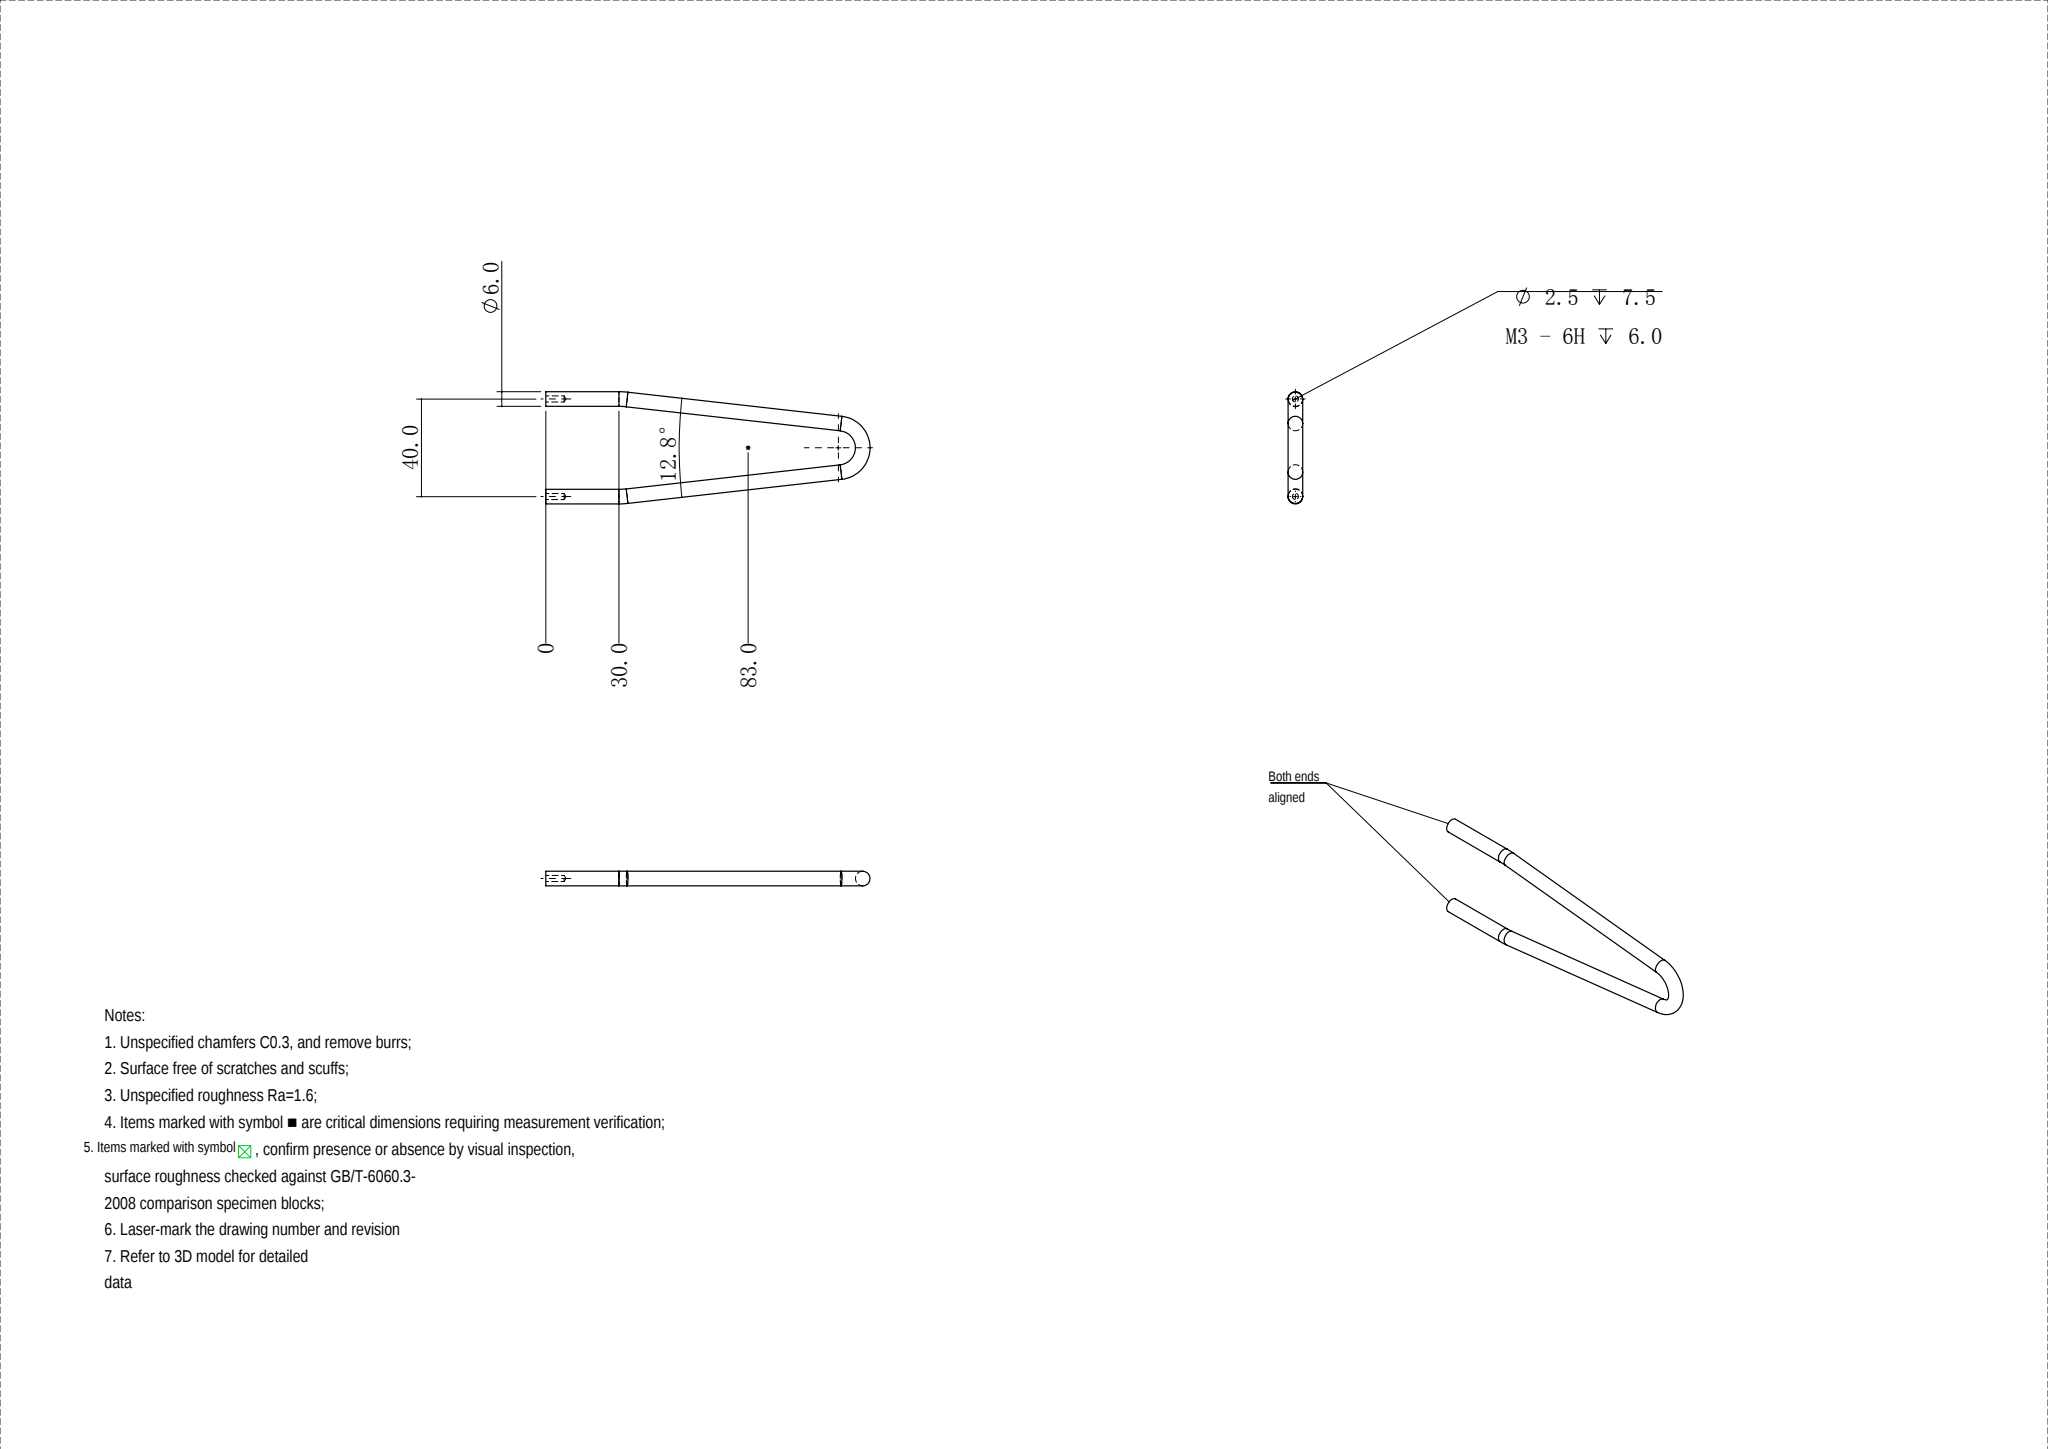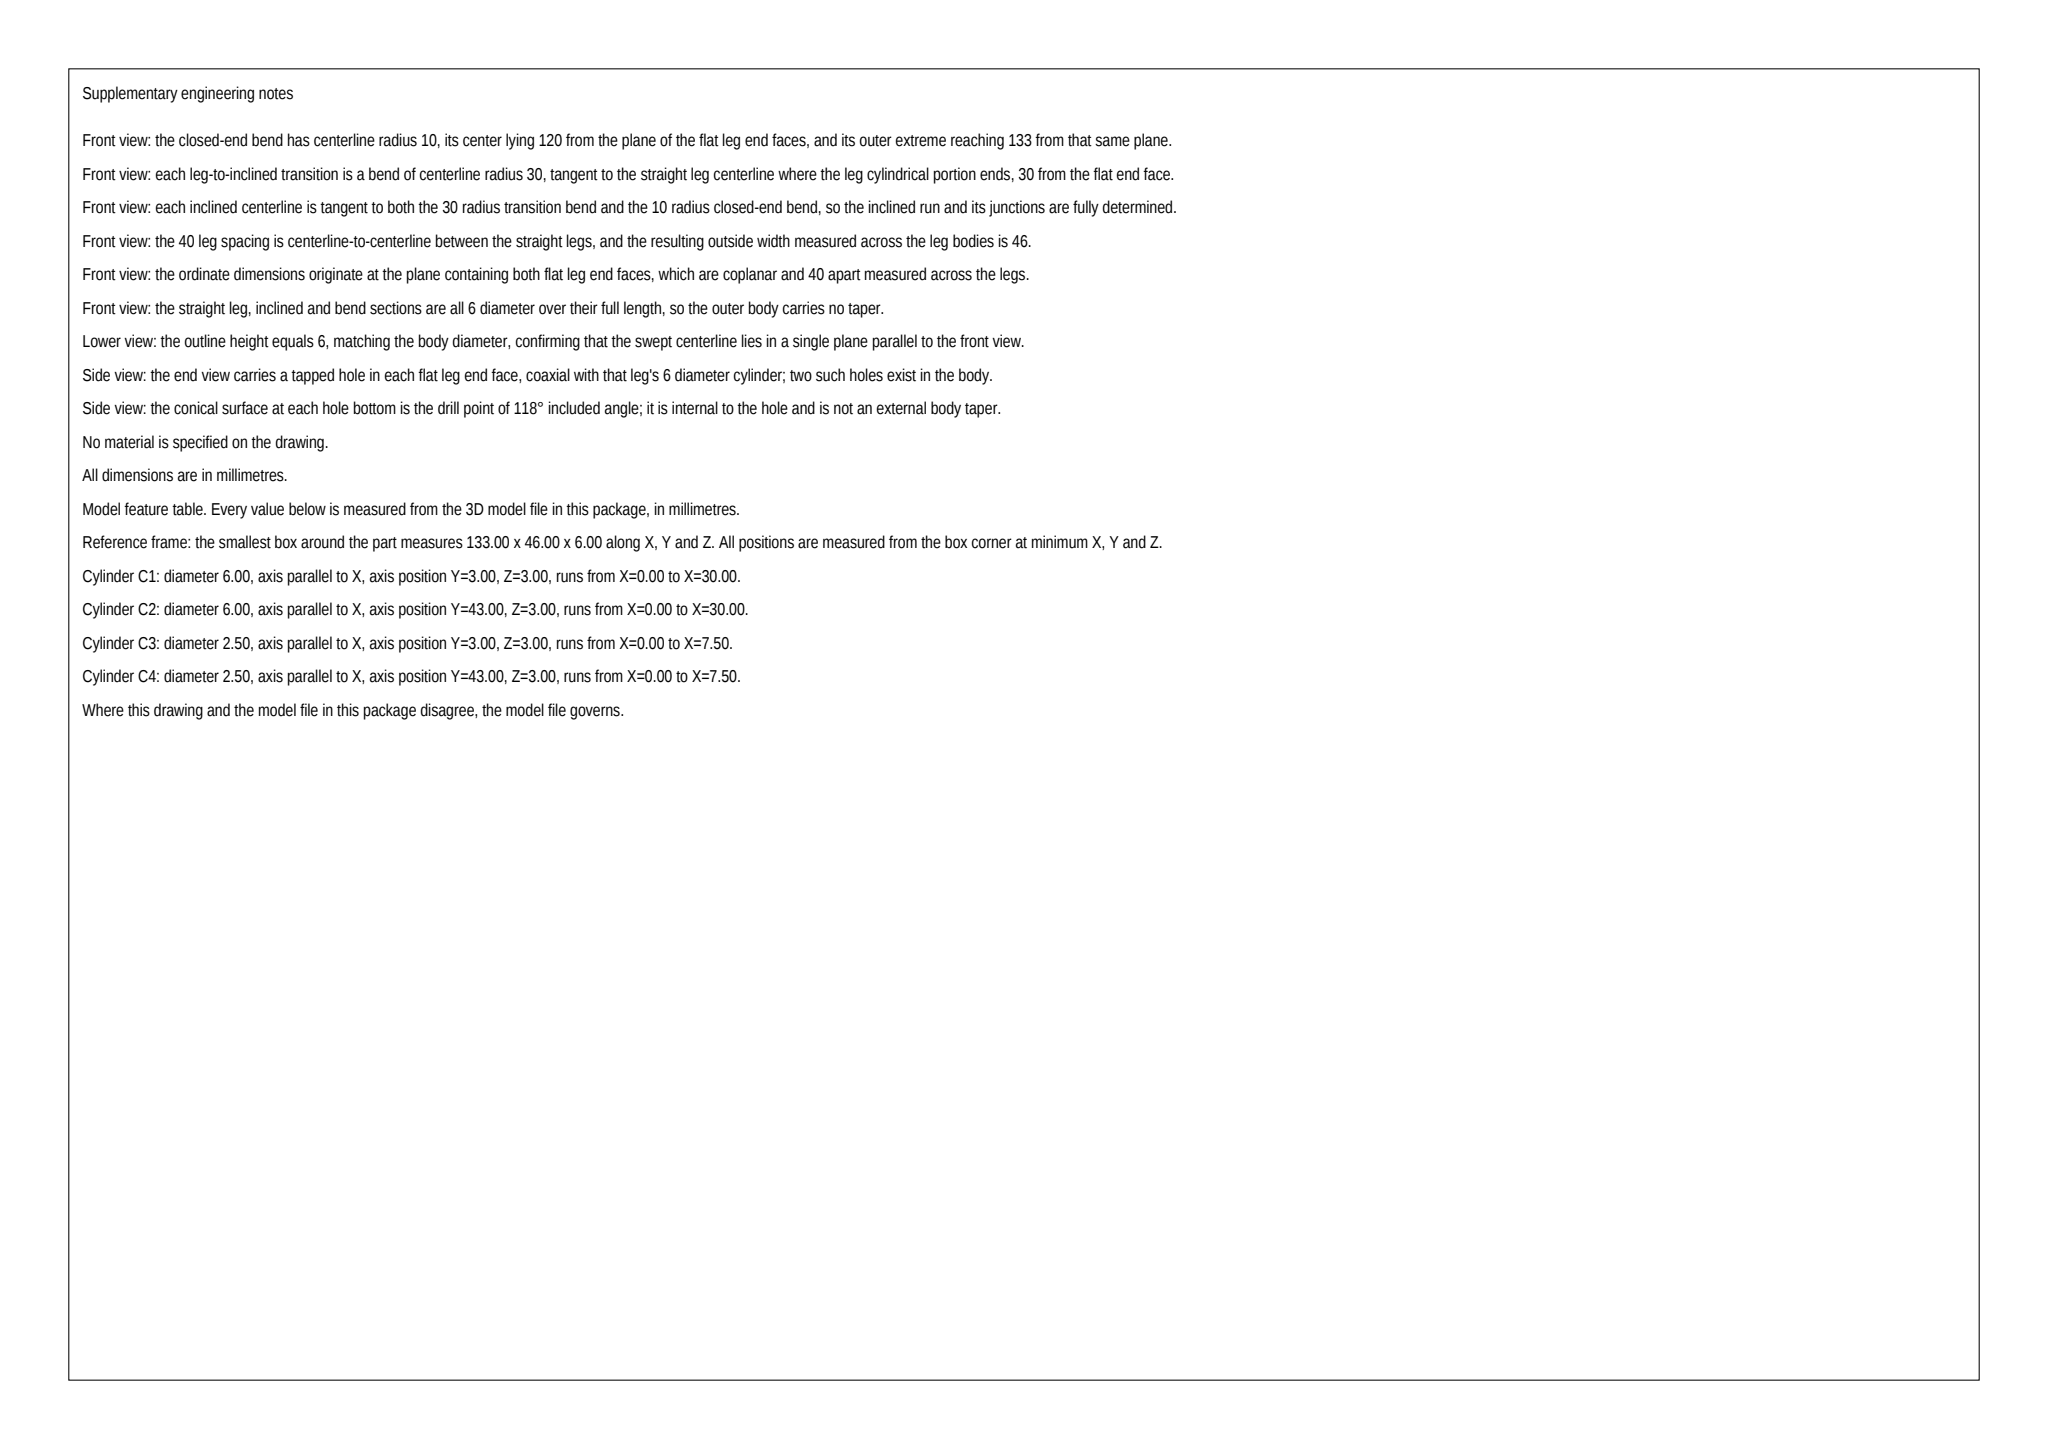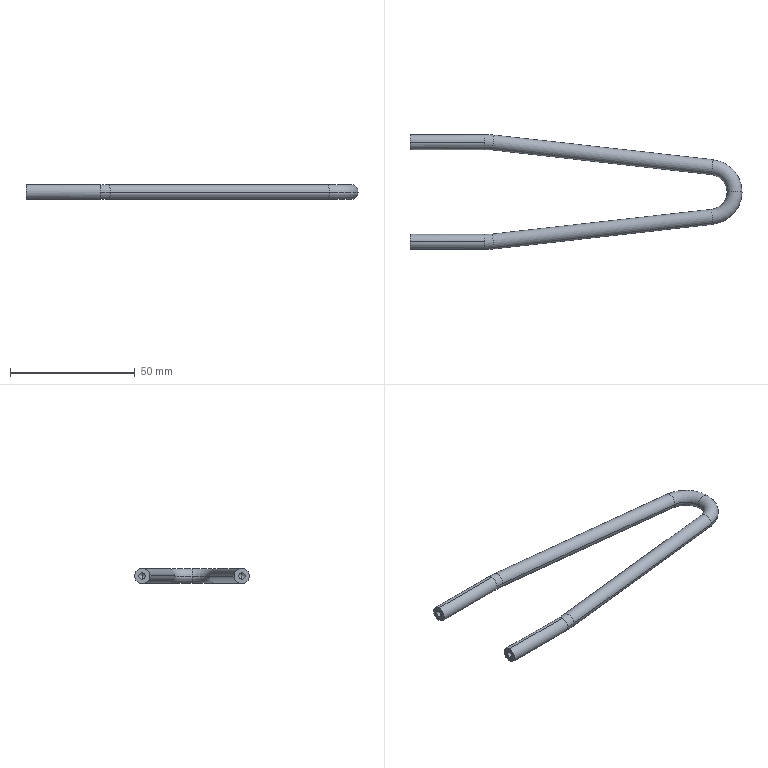Part | SolidWorks | mm | 1 solid | 26 faces | box 133 x 46 x 6 mm | volume 7630 mm3 | cylinder 12 | torus 8 | cone 4 | plane 2 | commonest cylinder face diameters 6 x8 2.5 x4
Drawing notes:
2X Ø2.5 DP 7.5, M3 - 6H DP 6.0 | from the solid: cylinders dia 2.5 axis x at y=3.05 and y=43.05, len 7.5, count 2 each (one per leg end)
Ø2.5/M3 HOLES COAX W/ Ø6.0 LEGS, IN END FACES AT STA 0 | from the solid: Ø2.5 holes share y=3.05/43.05, z=3.0 with Ø6.0 leg cylinders; axis plane x=0.0 end faces
40.0 IS CL-TO-CL OF Ø6.0 LEGS | from the solid: Ø6.0 leg axes at y=3.05 and y=43.05 -> 40.0 between centerlines
2X R30 TAN AT STA 30.0; 88.43 STRAIGHT TO R10 TANGENT | from the solid: Ø6.0 straight legs len 30.0 from x=0; angled Ø6.0 cylinders len 88.43 (y=3.24, y=32.99)
build123d program:
from build123d import *

# Parameters (mm, degrees)
SWEEP1_PROFILE_R      = 3
M3_TAPPED_HOLE1_D     = 2.5
M3_TAPPED_HOLE1_DEPTH = 7.5
M3_TAPPED_HOLE1_TIP   = 0.7511


with BuildPart() as part:
    # Sweep1: sweep along a curve in space
    with BuildLine() as sweep1_path:
        Line((0, 0, 0), (30, 0, 0))
        ThreePointArc((30, 0, 0), (31.68, -0.04706, 0), (33.354, -0.1881, 0))
        Line((33.354, -0.1881, 0), (121.118, -10.063, 0))
        ThreePointArc((121.118, -10.063, 0), (130, -20, 0), (121.118, -29.937, 0))
        Line((33.354, -39.812, 0), (121.118, -29.937, 0))
        ThreePointArc((30, -40, 0), (31.68, -39.953, 0), (33.354, -39.812, 0))
        Line((0, -40, 0), (30, -40, 0))
    # Sweep1 profile (on start of the path) → Sweep1 (sweep)
    with BuildSketch(Plane(origin=(0, 0, 0), x_dir=(0, 0, 1), z_dir=(1, 0, 0))):
        Circle(SWEEP1_PROFILE_R)
    sweep(path=sweep1_path.line)

    # M3 Tapped Hole1
    with Locations(Plane.ZY):
        with Locations((0, 0), (0, -40)):
            Hole(M3_TAPPED_HOLE1_D / 2, depth=M3_TAPPED_HOLE1_DEPTH)
            with Locations((0, 0, -(M3_TAPPED_HOLE1_DEPTH + M3_TAPPED_HOLE1_TIP / 2))):  # 118° drill point
                Cone(0, M3_TAPPED_HOLE1_D / 2, M3_TAPPED_HOLE1_TIP, mode=Mode.SUBTRACT)


solid = part.part
STEP:
#1=CARTESIAN_POINT('',(33.019,-3.169,0.));
#2=VERTEX_POINT('',#1);
#3=CARTESIAN_POINT('',(33.69,2.793,0.));
#4=VERTEX_POINT('',#3);
#5=CARTESIAN_POINT('',(33.354,-0.1881,0.));
#6=DIRECTION('',(-0.9937,0.1118,0.));
#7=DIRECTION('',(0.,0.,-1.));
#8=AXIS2_PLACEMENT_3D('',#5,#6,#7);
#9=CIRCLE('',#8,3.);
#10=EDGE_CURVE('',#2,#4,#9,.T.);
#11=ORIENTED_EDGE('',*,*,#10,.T.);
#12=CARTESIAN_POINT('',(30.,3.,0.));
#13=VERTEX_POINT('',#12);
#14=CARTESIAN_POINT('',(30.,-30.,0.));
#15=DIRECTION('',(0.,-0.,1.));
#16=DIRECTION('',(0.,-1.,-0.));
#17=AXIS2_PLACEMENT_3D('',#14,#15,#16);
#18=CIRCLE('',#17,33.);
#19=EDGE_CURVE('',#4,#13,#18,.T.);
#20=ORIENTED_EDGE('',*,*,#19,.T.);
#21=CARTESIAN_POINT('',(30.,0.,3.));
#22=VERTEX_POINT('',#21);
#23=CARTESIAN_POINT('',(30.,0.,0.));
#24=DIRECTION('',(-1.,-0.,0.));
#25=DIRECTION('',(0.,0.,-1.));
#26=AXIS2_PLACEMENT_3D('',#23,#24,#25);
#27=CIRCLE('',#26,3.);
#28=EDGE_CURVE('',#22,#13,#27,.T.);
#29=ORIENTED_EDGE('',*,*,#28,.F.);
#30=CARTESIAN_POINT('',(30.,-3.,0.));
#31=VERTEX_POINT('',#30);
#32=CARTESIAN_POINT('',(30.,0.,0.));
#33=DIRECTION('',(-1.,-0.,0.));
#34=DIRECTION('',(0.,0.,-1.));
#35=AXIS2_PLACEMENT_3D('',#32,#33,#34);
#36=CIRCLE('',#35,3.);
#37=EDGE_CURVE('',#31,#22,#36,.T.);
#38=ORIENTED_EDGE('',*,*,#37,.F.);
#39=CARTESIAN_POINT('',(30.,-30.,0.));
#40=DIRECTION('',(0.,-0.,1.));
#41=DIRECTION('',(0.,-1.,-0.));
#42=AXIS2_PLACEMENT_3D('',#39,#40,#41);
#43=CIRCLE('',#42,27.);
#44=EDGE_CURVE('',#2,#31,#43,.T.);
#45=ORIENTED_EDGE('',*,*,#44,.F.);
#46=EDGE_LOOP('',(#11,#20,#29,#38,#45));
#47=FACE_OUTER_BOUND('',#46,.T.);
#48=CARTESIAN_POINT('',(30.,-30.,0.));
#49=DIRECTION('',(0.,-0.,1.));
#50=DIRECTION('',(0.,-1.,-0.));
#51=AXIS2_PLACEMENT_3D('',#48,#49,#50);
#52=TOROIDAL_SURFACE('',#51,30.,3.);
#53=ADVANCED_FACE('',(#47),#52,.T.);
#54=CARTESIAN_POINT('',(133.,-20.,0.));
#55=VERTEX_POINT('',#54);
#56=CARTESIAN_POINT('',(127.,-20.,-0.));
#57=VERTEX_POINT('',#56);
#58=CARTESIAN_POINT('',(130.,-20.,0.));
#59=DIRECTION('',(0.,-1.,0.));
#60=DIRECTION('',(0.,0.,-1.));
#61=AXIS2_PLACEMENT_3D('',#58,#59,#60);
#62=CIRCLE('',#61,3.);
#63=EDGE_CURVE('',#55,#57,#62,.T.);
#64=ORIENTED_EDGE('',*,*,#63,.F.);
#65=CARTESIAN_POINT('',(121.454,-7.082,0.));
#66=VERTEX_POINT('',#65);
#67=CARTESIAN_POINT('',(120.,-20.,0.));
#68=DIRECTION('',(0.,0.,1.));
#69=DIRECTION('',(1.,0.,0.));
#70=AXIS2_PLACEMENT_3D('',#67,#68,#69);
#71=CIRCLE('',#70,13.);
#72=EDGE_CURVE('',#55,#66,#71,.T.);
#73=ORIENTED_EDGE('',*,*,#72,.T.);
#74=CARTESIAN_POINT('',(120.783,-13.044,0.));
#75=VERTEX_POINT('',#74);
#76=CARTESIAN_POINT('',(121.118,-10.063,0.));
#77=DIRECTION('',(-0.9937,0.1118,0.));
#78=DIRECTION('',(0.,0.,-1.));
#79=AXIS2_PLACEMENT_3D('',#76,#77,#78);
#80=CIRCLE('',#79,3.);
#81=EDGE_CURVE('',#75,#66,#80,.T.);
#82=ORIENTED_EDGE('',*,*,#81,.F.);
#83=CARTESIAN_POINT('',(120.,-20.,-0.));
#84=DIRECTION('',(0.,0.,1.));
#85=DIRECTION('',(1.,0.,0.));
#86=AXIS2_PLACEMENT_3D('',#83,#84,#85);
#87=CIRCLE('',#86,7.);
#88=EDGE_CURVE('',#57,#75,#87,.T.);
#89=ORIENTED_EDGE('',*,*,#88,.F.);
#90=EDGE_LOOP('',(#64,#73,#82,#89));
#91=FACE_OUTER_BOUND('',#90,.T.);
#92=CARTESIAN_POINT('',(120.,-20.,0.));
#93=DIRECTION('',(0.,0.,1.));
#94=DIRECTION('',(1.,0.,0.));
#95=AXIS2_PLACEMENT_3D('',#92,#93,#94);
#96=TOROIDAL_SURFACE('',#95,10.,3.);
#97=ADVANCED_FACE('',(#91),#96,.T.);
#98=CARTESIAN_POINT('',(30.,-40.,3.));
#99=VERTEX_POINT('',#98);
#100=CARTESIAN_POINT('',(30.,-43.,0.));
#101=VERTEX_POINT('',#100);
#102=CARTESIAN_POINT('',(30.,-40.,-0.));
#103=DIRECTION('',(1.,0.,-0.));
#104=DIRECTION('',(-0.,0.,-1.));
#105=AXIS2_PLACEMENT_3D('',#102,#103,#104);
#106=CIRCLE('',#105,3.);
#107=EDGE_CURVE('',#99,#101,#106,.T.);
#108=ORIENTED_EDGE('',*,*,#107,.T.);
#109=CARTESIAN_POINT('',(33.69,-42.793,0.));
#110=VERTEX_POINT('',#109);
#111=CARTESIAN_POINT('',(30.,-10.,0.));
#112=DIRECTION('',(0.,-0.,1.));
#113=DIRECTION('',(1.,0.,-0.));
#114=AXIS2_PLACEMENT_3D('',#111,#112,#113);
#115=CIRCLE('',#114,33.);
#116=EDGE_CURVE('',#101,#110,#115,.T.);
#117=ORIENTED_EDGE('',*,*,#116,.T.);
#118=CARTESIAN_POINT('',(33.019,-36.831,0.));
#119=VERTEX_POINT('',#118);
#120=CARTESIAN_POINT('',(33.354,-39.812,0.));
#121=DIRECTION('',(0.9937,0.1118,-0.));
#122=DIRECTION('',(0.,0.,-1.));
#123=AXIS2_PLACEMENT_3D('',#120,#121,#122);
#124=CIRCLE('',#123,3.);
#125=EDGE_CURVE('',#119,#110,#124,.T.);
#126=ORIENTED_EDGE('',*,*,#125,.F.);
#127=CARTESIAN_POINT('',(30.,-37.,0.));
#128=VERTEX_POINT('',#127);
#129=CARTESIAN_POINT('',(30.,-10.,0.));
#130=DIRECTION('',(0.,-0.,1.));
#131=DIRECTION('',(1.,0.,-0.));
#132=AXIS2_PLACEMENT_3D('',#129,#130,#131);
#133=CIRCLE('',#132,27.);
#134=EDGE_CURVE('',#128,#119,#133,.T.);
#135=ORIENTED_EDGE('',*,*,#134,.F.);
#136=CARTESIAN_POINT('',(30.,-40.,-0.));
#137=DIRECTION('',(1.,0.,-0.));
#138=DIRECTION('',(-0.,0.,-1.));
#139=AXIS2_PLACEMENT_3D('',#136,#137,#138);
#140=CIRCLE('',#139,3.);
#141=EDGE_CURVE('',#128,#99,#140,.T.);
#142=ORIENTED_EDGE('',*,*,#141,.T.);
#143=EDGE_LOOP('',(#108,#117,#126,#135,#142));
#144=FACE_OUTER_BOUND('',#143,.T.);
#145=CARTESIAN_POINT('',(30.,-10.,0.));
#146=DIRECTION('',(0.,-0.,1.));
#147=DIRECTION('',(1.,0.,-0.));
#148=AXIS2_PLACEMENT_3D('',#145,#146,#147);
#149=TOROIDAL_SURFACE('',#148,30.,3.);
#150=ADVANCED_FACE('',(#144),#149,.T.);
#151=CARTESIAN_POINT('',(120.783,-26.956,0.));
#152=VERTEX_POINT('',#151);
#153=CARTESIAN_POINT('',(121.454,-32.918,0.));
#154=VERTEX_POINT('',#153);
#155=CARTESIAN_POINT('',(121.118,-29.937,0.));
#156=DIRECTION('',(0.9937,0.1118,0.));
#157=DIRECTION('',(0.,0.,-1.));
#158=AXIS2_PLACEMENT_3D('',#155,#156,#157);
#159=CIRCLE('',#158,3.);
#160=EDGE_CURVE('',#152,#154,#159,.T.);
#161=ORIENTED_EDGE('',*,*,#160,.T.);
#162=CARTESIAN_POINT('',(120.,-20.,0.));
#163=DIRECTION('',(0.,0.,1.));
#164=DIRECTION('',(1.,0.,0.));
#165=AXIS2_PLACEMENT_3D('',#162,#163,#164);
#166=CIRCLE('',#165,13.);
#167=EDGE_CURVE('',#154,#55,#166,.T.);
#168=ORIENTED_EDGE('',*,*,#167,.T.);
#169=ORIENTED_EDGE('',*,*,#63,.T.);
#170=CARTESIAN_POINT('',(120.,-20.,-0.));
#171=DIRECTION('',(0.,0.,1.));
#172=DIRECTION('',(1.,0.,0.));
#173=AXIS2_PLACEMENT_3D('',#170,#171,#172);
#174=CIRCLE('',#173,7.);
#175=EDGE_CURVE('',#152,#57,#174,.T.);
#176=ORIENTED_EDGE('',*,*,#175,.F.);
#177=EDGE_LOOP('',(#161,#168,#169,#176));
#178=FACE_OUTER_BOUND('',#177,.T.);
#179=CARTESIAN_POINT('',(120.,-20.,0.));
#180=DIRECTION('',(0.,0.,1.));
#181=DIRECTION('',(1.,0.,0.));
#182=AXIS2_PLACEMENT_3D('',#179,#180,#181);
#183=TOROIDAL_SURFACE('',#182,10.,3.);
#184=ADVANCED_FACE('',(#178),#183,.T.);
#185=CARTESIAN_POINT('',(7.5,0.,-1.25));
#186=VERTEX_POINT('',#185);
#187=CARTESIAN_POINT('',(7.5,0.,1.25));
#188=VERTEX_POINT('',#187);
#189=CARTESIAN_POINT('',(7.5,0.,0.));
#190=DIRECTION('',(-1.,0.,0.));
#191=DIRECTION('',(0.,0.,1.));
#192=AXIS2_PLACEMENT_3D('',#189,#190,#191);
#193=CIRCLE('',#192,1.25);
#194=EDGE_CURVE('',#186,#188,#193,.T.);
#195=ORIENTED_EDGE('',*,*,#194,.F.);
#196=CARTESIAN_POINT('',(-0.,0.,-1.25));
#197=VERTEX_POINT('',#196);
#198=CARTESIAN_POINT('',(0.,0.,-1.25));
#199=DIRECTION('',(-1.,0.,0.));
#200=VECTOR('',#199,1000.);
#201=LINE('',#198,#200);
#202=EDGE_CURVE('',#186,#197,#201,.T.);
#203=ORIENTED_EDGE('',*,*,#202,.T.);
#204=CARTESIAN_POINT('',(-0.,0.,1.25));
#205=VERTEX_POINT('',#204);
#206=CARTESIAN_POINT('',(-0.,0.,0.));
#207=DIRECTION('',(-1.,0.,0.));
#208=DIRECTION('',(0.,0.,1.));
#209=AXIS2_PLACEMENT_3D('',#206,#207,#208);
#210=CIRCLE('',#209,1.25);
#211=EDGE_CURVE('',#197,#205,#210,.T.);
#212=ORIENTED_EDGE('',*,*,#211,.T.);
#213=CARTESIAN_POINT('',(0.,0.,1.25));
#214=DIRECTION('',(-1.,0.,0.));
#215=VECTOR('',#214,1000.);
#216=LINE('',#213,#215);
#217=EDGE_CURVE('',#188,#205,#216,.T.);
#218=ORIENTED_EDGE('',*,*,#217,.F.);
#219=EDGE_LOOP('',(#195,#203,#212,#218));
#220=FACE_OUTER_BOUND('',#219,.T.);
#221=CARTESIAN_POINT('',(0.,0.,0.));
#222=DIRECTION('',(-1.,0.,0.));
#223=DIRECTION('',(0.,0.,1.));
#224=AXIS2_PLACEMENT_3D('',#221,#222,#223);
#225=CYLINDRICAL_SURFACE('',#224,1.25);
#226=ADVANCED_FACE('',(#220),#225,.F.);
#227=CARTESIAN_POINT('',(8.251,-0.,0.));
#228=VERTEX_POINT('',#227);
#229=CARTESIAN_POINT('',(7.5,0.,1.25));
#230=DIRECTION('',(-0.515,0.,0.8572));
#231=VECTOR('',#230,1000.);
#232=LINE('',#229,#231);
#233=EDGE_CURVE('',#228,#188,#232,.T.);
#234=ORIENTED_EDGE('',*,*,#233,.F.);
#235=CARTESIAN_POINT('',(7.5,0.,-1.25));
#236=DIRECTION('',(-0.515,0.,-0.8572));
#237=VECTOR('',#236,1000.);
#238=LINE('',#235,#237);
#239=EDGE_CURVE('',#228,#186,#238,.T.);
#240=ORIENTED_EDGE('',*,*,#239,.T.);
#241=ORIENTED_EDGE('',*,*,#194,.T.);
#242=EDGE_LOOP('',(#234,#240,#241));
#243=FACE_OUTER_BOUND('',#242,.T.);
#244=CARTESIAN_POINT('',(7.5,0.,0.));
#245=DIRECTION('',(-1.,0.,0.));
#246=DIRECTION('',(0.,0.,1.));
#247=AXIS2_PLACEMENT_3D('',#244,#245,#246);
#248=CONICAL_SURFACE('',#247,1.25,1.03);
#249=ADVANCED_FACE('',(#243),#248,.F.);
#250=CARTESIAN_POINT('',(7.5,-40.,-1.25));
#251=VERTEX_POINT('',#250);
#252=CARTESIAN_POINT('',(7.5,-40.,1.25));
#253=VERTEX_POINT('',#252);
#254=CARTESIAN_POINT('',(7.5,-40.,-0.));
#255=DIRECTION('',(-1.,0.,0.));
#256=DIRECTION('',(0.,0.,1.));
#257=AXIS2_PLACEMENT_3D('',#254,#255,#256);
#258=CIRCLE('',#257,1.25);
#259=EDGE_CURVE('',#251,#253,#258,.T.);
#260=ORIENTED_EDGE('',*,*,#259,.F.);
#261=CARTESIAN_POINT('',(-0.,-40.,-1.25));
#262=VERTEX_POINT('',#261);
#263=CARTESIAN_POINT('',(0.,-40.,-1.25));
#264=DIRECTION('',(-1.,0.,0.));
#265=VECTOR('',#264,1000.);
#266=LINE('',#263,#265);
#267=EDGE_CURVE('',#251,#262,#266,.T.);
#268=ORIENTED_EDGE('',*,*,#267,.T.);
#269=CARTESIAN_POINT('',(-0.,-40.,1.25));
#270=VERTEX_POINT('',#269);
#271=CARTESIAN_POINT('',(-0.,-40.,-0.));
#272=DIRECTION('',(-1.,0.,0.));
#273=DIRECTION('',(0.,0.,1.));
#274=AXIS2_PLACEMENT_3D('',#271,#272,#273);
#275=CIRCLE('',#274,1.25);
#276=EDGE_CURVE('',#262,#270,#275,.T.);
#277=ORIENTED_EDGE('',*,*,#276,.T.);
#278=CARTESIAN_POINT('',(0.,-40.,1.25));
#279=DIRECTION('',(-1.,0.,0.));
#280=VECTOR('',#279,1000.);
#281=LINE('',#278,#280);
#282=EDGE_CURVE('',#253,#270,#281,.T.);
#283=ORIENTED_EDGE('',*,*,#282,.F.);
#284=EDGE_LOOP('',(#260,#268,#277,#283));
#285=FACE_OUTER_BOUND('',#284,.T.);
#286=CARTESIAN_POINT('',(0.,-40.,-0.));
#287=DIRECTION('',(-1.,0.,0.));
#288=DIRECTION('',(0.,0.,1.));
#289=AXIS2_PLACEMENT_3D('',#286,#287,#288);
#290=CYLINDRICAL_SURFACE('',#289,1.25);
#291=ADVANCED_FACE('',(#285),#290,.F.);
#292=CARTESIAN_POINT('',(8.251,-40.,-0.));
#293=VERTEX_POINT('',#292);
#294=CARTESIAN_POINT('',(7.5,-40.,1.25));
#295=DIRECTION('',(-0.515,0.,0.8572));
#296=VECTOR('',#295,1000.);
#297=LINE('',#294,#296);
#298=EDGE_CURVE('',#293,#253,#297,.T.);
#299=ORIENTED_EDGE('',*,*,#298,.F.);
#300=CARTESIAN_POINT('',(7.5,-40.,-1.25));
#301=DIRECTION('',(-0.515,0.,-0.8572));
#302=VECTOR('',#301,1000.);
#303=LINE('',#300,#302);
#304=EDGE_CURVE('',#293,#251,#303,.T.);
#305=ORIENTED_EDGE('',*,*,#304,.T.);
#306=ORIENTED_EDGE('',*,*,#259,.T.);
#307=EDGE_LOOP('',(#299,#305,#306));
#308=FACE_OUTER_BOUND('',#307,.T.);
#309=CARTESIAN_POINT('',(7.5,-40.,-0.));
#310=DIRECTION('',(-1.,0.,0.));
#311=DIRECTION('',(0.,0.,1.));
#312=AXIS2_PLACEMENT_3D('',#309,#310,#311);
#313=CONICAL_SURFACE('',#312,1.25,1.03);
#314=ADVANCED_FACE('',(#308),#313,.F.);
#315=ORIENTED_EDGE('',*,*,#28,.T.);
#316=CARTESIAN_POINT('',(30.,0.,-3.));
#317=VERTEX_POINT('',#316);
#318=CARTESIAN_POINT('',(30.,0.,0.));
#319=DIRECTION('',(-1.,-0.,0.));
#320=DIRECTION('',(0.,0.,-1.));
#321=AXIS2_PLACEMENT_3D('',#318,#319,#320);
#322=CIRCLE('',#321,3.);
#323=EDGE_CURVE('',#13,#317,#322,.T.);
#324=ORIENTED_EDGE('',*,*,#323,.T.);
#325=CARTESIAN_POINT('',(-0.,0.,-3.));
#326=VERTEX_POINT('',#325);
#327=CARTESIAN_POINT('',(30.,0.,-3.));
#328=DIRECTION('',(-1.,0.,0.));
#329=VECTOR('',#328,1000.);
#330=LINE('',#327,#329);
#331=EDGE_CURVE('',#317,#326,#330,.T.);
#332=ORIENTED_EDGE('',*,*,#331,.T.);
#333=CARTESIAN_POINT('',(0.,0.,3.));
#334=VERTEX_POINT('',#333);
#335=CARTESIAN_POINT('',(0.,0.,0.));
#336=DIRECTION('',(-1.,-0.,0.));
#337=DIRECTION('',(-0.,0.,-1.));
#338=AXIS2_PLACEMENT_3D('',#335,#336,#337);
#339=CIRCLE('',#338,3.);
#340=EDGE_CURVE('',#334,#326,#339,.T.);
#341=ORIENTED_EDGE('',*,*,#340,.F.);
#342=CARTESIAN_POINT('',(30.,0.,3.));
#343=DIRECTION('',(-1.,0.,0.));
#344=VECTOR('',#343,1000.);
#345=LINE('',#342,#344);
#346=EDGE_CURVE('',#22,#334,#345,.T.);
#347=ORIENTED_EDGE('',*,*,#346,.F.);
#348=EDGE_LOOP('',(#315,#324,#332,#341,#347));
#349=FACE_OUTER_BOUND('',#348,.T.);
#350=CARTESIAN_POINT('',(30.,0.,0.));
#351=DIRECTION('',(-1.,0.,0.));
#352=DIRECTION('',(0.,0.,1.));
#353=AXIS2_PLACEMENT_3D('',#350,#351,#352);
#354=CYLINDRICAL_SURFACE('',#353,3.);
#355=ADVANCED_FACE('',(#349),#354,.T.);
#356=ORIENTED_EDGE('',*,*,#81,.T.);
#357=CARTESIAN_POINT('',(121.454,-7.082,0.));
#358=DIRECTION('',(-0.9937,0.1118,-0.));
#359=VECTOR('',#358,1000.);
#360=LINE('',#357,#359);
#361=EDGE_CURVE('',#66,#4,#360,.T.);
#362=ORIENTED_EDGE('',*,*,#361,.T.);
#363=ORIENTED_EDGE('',*,*,#10,.F.);
#364=CARTESIAN_POINT('',(120.783,-13.044,0.));
#365=DIRECTION('',(-0.9937,0.1118,-0.));
#366=VECTOR('',#365,1000.);
#367=LINE('',#364,#366);
#368=EDGE_CURVE('',#75,#2,#367,.T.);
#369=ORIENTED_EDGE('',*,*,#368,.F.);
#370=EDGE_LOOP('',(#356,#362,#363,#369));
#371=FACE_OUTER_BOUND('',#370,.T.);
#372=CARTESIAN_POINT('',(121.118,-10.063,0.));
#373=DIRECTION('',(-0.9937,0.1118,-0.));
#374=DIRECTION('',(-0.1118,-0.9937,0.));
#375=AXIS2_PLACEMENT_3D('',#372,#373,#374);
#376=CYLINDRICAL_SURFACE('',#375,3.);
#377=ADVANCED_FACE('',(#371),#376,.T.);
#378=ORIENTED_EDGE('',*,*,#167,.F.);
#379=CARTESIAN_POINT('',(121.118,-29.937,0.));
#380=DIRECTION('',(0.9937,0.1118,0.));
#381=DIRECTION('',(0.,0.,-1.));
#382=AXIS2_PLACEMENT_3D('',#379,#380,#381);
#383=CIRCLE('',#382,3.);
#384=EDGE_CURVE('',#154,#152,#383,.T.);
#385=ORIENTED_EDGE('',*,*,#384,.T.);
#386=ORIENTED_EDGE('',*,*,#175,.T.);
#387=CARTESIAN_POINT('',(130.,-20.,0.));
#388=DIRECTION('',(0.,-1.,0.));
#389=DIRECTION('',(0.,0.,-1.));
#390=AXIS2_PLACEMENT_3D('',#387,#388,#389);
#391=CIRCLE('',#390,3.);
#392=EDGE_CURVE('',#57,#55,#391,.T.);
#393=ORIENTED_EDGE('',*,*,#392,.T.);
#394=EDGE_LOOP('',(#378,#385,#386,#393));
#395=FACE_OUTER_BOUND('',#394,.T.);
#396=CARTESIAN_POINT('',(120.,-20.,0.));
#397=DIRECTION('',(0.,0.,1.));
#398=DIRECTION('',(1.,0.,0.));
#399=AXIS2_PLACEMENT_3D('',#396,#397,#398);
#400=TOROIDAL_SURFACE('',#399,10.,3.);
#401=ADVANCED_FACE('',(#395),#400,.T.);
#402=ORIENTED_EDGE('',*,*,#125,.T.);
#403=CARTESIAN_POINT('',(33.69,-42.793,0.));
#404=DIRECTION('',(0.9937,0.1118,0.));
#405=VECTOR('',#404,1000.);
#406=LINE('',#403,#405);
#407=EDGE_CURVE('',#110,#154,#406,.T.);
#408=ORIENTED_EDGE('',*,*,#407,.T.);
#409=ORIENTED_EDGE('',*,*,#160,.F.);
#410=CARTESIAN_POINT('',(33.019,-36.831,0.));
#411=DIRECTION('',(0.9937,0.1118,0.));
#412=VECTOR('',#411,1000.);
#413=LINE('',#410,#412);
#414=EDGE_CURVE('',#119,#152,#413,.T.);
#415=ORIENTED_EDGE('',*,*,#414,.F.);
#416=EDGE_LOOP('',(#402,#408,#409,#415));
#417=FACE_OUTER_BOUND('',#416,.T.);
#418=CARTESIAN_POINT('',(33.354,-39.812,0.));
#419=DIRECTION('',(0.9937,0.1118,0.));
#420=DIRECTION('',(-0.1118,0.9937,0.));
#421=AXIS2_PLACEMENT_3D('',#418,#419,#420);
#422=CYLINDRICAL_SURFACE('',#421,3.);
#423=ADVANCED_FACE('',(#417),#422,.T.);
#424=CARTESIAN_POINT('',(-0.,-40.,-3.));
#425=VERTEX_POINT('',#424);
#426=CARTESIAN_POINT('',(0.,-40.,3.));
#427=VERTEX_POINT('',#426);
#428=CARTESIAN_POINT('',(0.,-40.,-0.));
#429=DIRECTION('',(1.,0.,-0.));
#430=DIRECTION('',(-0.,0.,-1.));
#431=AXIS2_PLACEMENT_3D('',#428,#429,#430);
#432=CIRCLE('',#431,3.);
#433=EDGE_CURVE('',#425,#427,#432,.T.);
#434=ORIENTED_EDGE('',*,*,#433,.T.);
#435=CARTESIAN_POINT('',(0.,-40.,3.));
#436=DIRECTION('',(1.,0.,-0.));
#437=VECTOR('',#436,1000.);
#438=LINE('',#435,#437);
#439=EDGE_CURVE('',#427,#99,#438,.T.);
#440=ORIENTED_EDGE('',*,*,#439,.T.);
#441=ORIENTED_EDGE('',*,*,#141,.F.);
#442=CARTESIAN_POINT('',(30.,-40.,-3.));
#443=VERTEX_POINT('',#442);
#444=CARTESIAN_POINT('',(30.,-40.,-0.));
#445=DIRECTION('',(1.,0.,-0.));
#446=DIRECTION('',(-0.,0.,-1.));
#447=AXIS2_PLACEMENT_3D('',#444,#445,#446);
#448=CIRCLE('',#447,3.);
#449=EDGE_CURVE('',#443,#128,#448,.T.);
#450=ORIENTED_EDGE('',*,*,#449,.F.);
#451=CARTESIAN_POINT('',(-0.,-40.,-3.));
#452=DIRECTION('',(1.,0.,-0.));
#453=VECTOR('',#452,1000.);
#454=LINE('',#451,#453);
#455=EDGE_CURVE('',#425,#443,#454,.T.);
#456=ORIENTED_EDGE('',*,*,#455,.F.);
#457=EDGE_LOOP('',(#434,#440,#441,#450,#456));
#458=FACE_OUTER_BOUND('',#457,.T.);
#459=CARTESIAN_POINT('',(0.,-40.,-0.));
#460=DIRECTION('',(1.,0.,-0.));
#461=DIRECTION('',(-0.,0.,-1.));
#462=AXIS2_PLACEMENT_3D('',#459,#460,#461);
#463=CYLINDRICAL_SURFACE('',#462,3.);
#464=ADVANCED_FACE('',(#458),#463,.T.);
#465=ORIENTED_EDGE('',*,*,#331,.F.);
#466=CARTESIAN_POINT('',(30.,0.,0.));
#467=DIRECTION('',(-1.,-0.,0.));
#468=DIRECTION('',(0.,0.,-1.));
#469=AXIS2_PLACEMENT_3D('',#466,#467,#468);
#470=CIRCLE('',#469,3.);
#471=EDGE_CURVE('',#317,#31,#470,.T.);
#472=ORIENTED_EDGE('',*,*,#471,.T.);
#473=ORIENTED_EDGE('',*,*,#37,.T.);
#474=ORIENTED_EDGE('',*,*,#346,.T.);
#475=CARTESIAN_POINT('',(0.,0.,0.));
#476=DIRECTION('',(-1.,-0.,0.));
#477=DIRECTION('',(-0.,0.,-1.));
#478=AXIS2_PLACEMENT_3D('',#475,#476,#477);
#479=CIRCLE('',#478,3.);
#480=EDGE_CURVE('',#326,#334,#479,.T.);
#481=ORIENTED_EDGE('',*,*,#480,.F.);
#482=EDGE_LOOP('',(#465,#472,#473,#474,#481));
#483=FACE_OUTER_BOUND('',#482,.T.);
#484=CARTESIAN_POINT('',(30.,0.,0.));
#485=DIRECTION('',(-1.,0.,0.));
#486=DIRECTION('',(0.,0.,1.));
#487=AXIS2_PLACEMENT_3D('',#484,#485,#486);
#488=CYLINDRICAL_SURFACE('',#487,3.);
#489=ADVANCED_FACE('',(#483),#488,.T.);
#490=ORIENTED_EDGE('',*,*,#19,.F.);
#491=CARTESIAN_POINT('',(33.354,-0.1881,0.));
#492=DIRECTION('',(-0.9937,0.1118,0.));
#493=DIRECTION('',(0.,0.,-1.));
#494=AXIS2_PLACEMENT_3D('',#491,#492,#493);
#495=CIRCLE('',#494,3.);
#496=EDGE_CURVE('',#4,#2,#495,.T.);
#497=ORIENTED_EDGE('',*,*,#496,.T.);
#498=ORIENTED_EDGE('',*,*,#44,.T.);
#499=ORIENTED_EDGE('',*,*,#471,.F.);
#500=ORIENTED_EDGE('',*,*,#323,.F.);
#501=EDGE_LOOP('',(#490,#497,#498,#499,#500));
#502=FACE_OUTER_BOUND('',#501,.T.);
#503=CARTESIAN_POINT('',(30.,-30.,0.));
#504=DIRECTION('',(0.,-0.,1.));
#505=DIRECTION('',(0.,-1.,-0.));
#506=AXIS2_PLACEMENT_3D('',#503,#504,#505);
#507=TOROIDAL_SURFACE('',#506,30.,3.);
#508=ADVANCED_FACE('',(#502),#507,.T.);
#509=ORIENTED_EDGE('',*,*,#361,.F.);
#510=CARTESIAN_POINT('',(121.118,-10.063,0.));
#511=DIRECTION('',(-0.9937,0.1118,0.));
#512=DIRECTION('',(0.,0.,-1.));
#513=AXIS2_PLACEMENT_3D('',#510,#511,#512);
#514=CIRCLE('',#513,3.);
#515=EDGE_CURVE('',#66,#75,#514,.T.);
#516=ORIENTED_EDGE('',*,*,#515,.T.);
#517=ORIENTED_EDGE('',*,*,#368,.T.);
#518=ORIENTED_EDGE('',*,*,#496,.F.);
#519=EDGE_LOOP('',(#509,#516,#517,#518));
#520=FACE_OUTER_BOUND('',#519,.T.);
#521=CARTESIAN_POINT('',(121.118,-10.063,0.));
#522=DIRECTION('',(-0.9937,0.1118,-0.));
#523=DIRECTION('',(-0.1118,-0.9937,0.));
#524=AXIS2_PLACEMENT_3D('',#521,#522,#523);
#525=CYLINDRICAL_SURFACE('',#524,3.);
#526=ADVANCED_FACE('',(#520),#525,.T.);
#527=ORIENTED_EDGE('',*,*,#72,.F.);
#528=ORIENTED_EDGE('',*,*,#392,.F.);
#529=ORIENTED_EDGE('',*,*,#88,.T.);
#530=ORIENTED_EDGE('',*,*,#515,.F.);
#531=EDGE_LOOP('',(#527,#528,#529,#530));
#532=FACE_OUTER_BOUND('',#531,.T.);
#533=CARTESIAN_POINT('',(120.,-20.,0.));
#534=DIRECTION('',(0.,0.,1.));
#535=DIRECTION('',(1.,0.,0.));
#536=AXIS2_PLACEMENT_3D('',#533,#534,#535);
#537=TOROIDAL_SURFACE('',#536,10.,3.);
#538=ADVANCED_FACE('',(#532),#537,.T.);
#539=ORIENTED_EDGE('',*,*,#407,.F.);
#540=CARTESIAN_POINT('',(33.354,-39.812,0.));
#541=DIRECTION('',(0.9937,0.1118,-0.));
#542=DIRECTION('',(0.,0.,-1.));
#543=AXIS2_PLACEMENT_3D('',#540,#541,#542);
#544=CIRCLE('',#543,3.);
#545=EDGE_CURVE('',#110,#119,#544,.T.);
#546=ORIENTED_EDGE('',*,*,#545,.T.);
#547=ORIENTED_EDGE('',*,*,#414,.T.);
#548=ORIENTED_EDGE('',*,*,#384,.F.);
#549=EDGE_LOOP('',(#539,#546,#547,#548));
#550=FACE_OUTER_BOUND('',#549,.T.);
#551=CARTESIAN_POINT('',(33.354,-39.812,0.));
#552=DIRECTION('',(0.9937,0.1118,0.));
#553=DIRECTION('',(-0.1118,0.9937,0.));
#554=AXIS2_PLACEMENT_3D('',#551,#552,#553);
#555=CYLINDRICAL_SURFACE('',#554,3.);
#556=ADVANCED_FACE('',(#550),#555,.T.);
#557=ORIENTED_EDGE('',*,*,#116,.F.);
#558=CARTESIAN_POINT('',(30.,-40.,-0.));
#559=DIRECTION('',(1.,0.,-0.));
#560=DIRECTION('',(-0.,0.,-1.));
#561=AXIS2_PLACEMENT_3D('',#558,#559,#560);
#562=CIRCLE('',#561,3.);
#563=EDGE_CURVE('',#101,#443,#562,.T.);
#564=ORIENTED_EDGE('',*,*,#563,.T.);
#565=ORIENTED_EDGE('',*,*,#449,.T.);
#566=ORIENTED_EDGE('',*,*,#134,.T.);
#567=ORIENTED_EDGE('',*,*,#545,.F.);
#568=EDGE_LOOP('',(#557,#564,#565,#566,#567));
#569=FACE_OUTER_BOUND('',#568,.T.);
#570=CARTESIAN_POINT('',(30.,-10.,0.));
#571=DIRECTION('',(0.,-0.,1.));
#572=DIRECTION('',(1.,0.,-0.));
#573=AXIS2_PLACEMENT_3D('',#570,#571,#572);
#574=TOROIDAL_SURFACE('',#573,30.,3.);
#575=ADVANCED_FACE('',(#569),#574,.T.);
#576=ORIENTED_EDGE('',*,*,#439,.F.);
#577=CARTESIAN_POINT('',(0.,-40.,-0.));
#578=DIRECTION('',(1.,0.,-0.));
#579=DIRECTION('',(-0.,0.,-1.));
#580=AXIS2_PLACEMENT_3D('',#577,#578,#579);
#581=CIRCLE('',#580,3.);
#582=EDGE_CURVE('',#427,#425,#581,.T.);
#583=ORIENTED_EDGE('',*,*,#582,.T.);
#584=ORIENTED_EDGE('',*,*,#455,.T.);
#585=ORIENTED_EDGE('',*,*,#563,.F.);
#586=ORIENTED_EDGE('',*,*,#107,.F.);
#587=EDGE_LOOP('',(#576,#583,#584,#585,#586));
#588=FACE_OUTER_BOUND('',#587,.T.);
#589=CARTESIAN_POINT('',(0.,-40.,-0.));
#590=DIRECTION('',(1.,0.,-0.));
#591=DIRECTION('',(-0.,0.,-1.));
#592=AXIS2_PLACEMENT_3D('',#589,#590,#591);
#593=CYLINDRICAL_SURFACE('',#592,3.);
#594=ADVANCED_FACE('',(#588),#593,.T.);
#595=CARTESIAN_POINT('',(-0.,0.,0.));
#596=DIRECTION('',(-1.,0.,0.));
#597=DIRECTION('',(0.,0.,1.));
#598=AXIS2_PLACEMENT_3D('',#595,#596,#597);
#599=CIRCLE('',#598,1.25);
#600=EDGE_CURVE('',#205,#197,#599,.T.);
#601=ORIENTED_EDGE('',*,*,#600,.F.);
#602=ORIENTED_EDGE('',*,*,#211,.F.);
#603=EDGE_LOOP('',(#601,#602));
#604=FACE_BOUND('',#603,.T.);
#605=ORIENTED_EDGE('',*,*,#340,.T.);
#606=ORIENTED_EDGE('',*,*,#480,.T.);
#607=EDGE_LOOP('',(#605,#606));
#608=FACE_OUTER_BOUND('',#607,.T.);
#609=CARTESIAN_POINT('',(0.,0.,0.));
#610=DIRECTION('',(-1.,-0.,0.));
#611=DIRECTION('',(-0.,0.,-1.));
#612=AXIS2_PLACEMENT_3D('',#609,#610,#611);
#613=PLANE('',#612);
#614=ADVANCED_FACE('',(#604,#608),#613,.T.);
#615=CARTESIAN_POINT('',(-0.,-40.,-0.));
#616=DIRECTION('',(-1.,0.,0.));
#617=DIRECTION('',(0.,0.,1.));
#618=AXIS2_PLACEMENT_3D('',#615,#616,#617);
#619=CIRCLE('',#618,1.25);
#620=EDGE_CURVE('',#270,#262,#619,.T.);
#621=ORIENTED_EDGE('',*,*,#620,.F.);
#622=ORIENTED_EDGE('',*,*,#276,.F.);
#623=EDGE_LOOP('',(#621,#622));
#624=FACE_BOUND('',#623,.T.);
#625=ORIENTED_EDGE('',*,*,#433,.F.);
#626=ORIENTED_EDGE('',*,*,#582,.F.);
#627=EDGE_LOOP('',(#625,#626));
#628=FACE_OUTER_BOUND('',#627,.T.);
#629=CARTESIAN_POINT('',(0.,-40.,-0.));
#630=DIRECTION('',(1.,0.,-0.));
#631=DIRECTION('',(-0.,0.,-1.));
#632=AXIS2_PLACEMENT_3D('',#629,#630,#631);
#633=PLANE('',#632);
#634=ADVANCED_FACE('',(#624,#628),#633,.F.);
#635=ORIENTED_EDGE('',*,*,#304,.F.);
#636=ORIENTED_EDGE('',*,*,#298,.T.);
#637=CARTESIAN_POINT('',(7.5,-40.,-0.));
#638=DIRECTION('',(-1.,0.,0.));
#639=DIRECTION('',(0.,0.,1.));
#640=AXIS2_PLACEMENT_3D('',#637,#638,#639);
#641=CIRCLE('',#640,1.25);
#642=EDGE_CURVE('',#253,#251,#641,.T.);
#643=ORIENTED_EDGE('',*,*,#642,.T.);
#644=EDGE_LOOP('',(#635,#636,#643));
#645=FACE_OUTER_BOUND('',#644,.T.);
#646=CARTESIAN_POINT('',(7.5,-40.,-0.));
#647=DIRECTION('',(-1.,0.,0.));
#648=DIRECTION('',(0.,0.,1.));
#649=AXIS2_PLACEMENT_3D('',#646,#647,#648);
#650=CONICAL_SURFACE('',#649,1.25,1.03);
#651=ADVANCED_FACE('',(#645),#650,.F.);
#652=ORIENTED_EDGE('',*,*,#267,.F.);
#653=ORIENTED_EDGE('',*,*,#642,.F.);
#654=ORIENTED_EDGE('',*,*,#282,.T.);
#655=ORIENTED_EDGE('',*,*,#620,.T.);
#656=EDGE_LOOP('',(#652,#653,#654,#655));
#657=FACE_OUTER_BOUND('',#656,.T.);
#658=CARTESIAN_POINT('',(0.,-40.,-0.));
#659=DIRECTION('',(-1.,0.,0.));
#660=DIRECTION('',(0.,0.,1.));
#661=AXIS2_PLACEMENT_3D('',#658,#659,#660);
#662=CYLINDRICAL_SURFACE('',#661,1.25);
#663=ADVANCED_FACE('',(#657),#662,.F.);
#664=ORIENTED_EDGE('',*,*,#239,.F.);
#665=ORIENTED_EDGE('',*,*,#233,.T.);
#666=CARTESIAN_POINT('',(7.5,0.,0.));
#667=DIRECTION('',(-1.,0.,0.));
#668=DIRECTION('',(0.,0.,1.));
#669=AXIS2_PLACEMENT_3D('',#666,#667,#668);
#670=CIRCLE('',#669,1.25);
#671=EDGE_CURVE('',#188,#186,#670,.T.);
#672=ORIENTED_EDGE('',*,*,#671,.T.);
#673=EDGE_LOOP('',(#664,#665,#672));
#674=FACE_OUTER_BOUND('',#673,.T.);
#675=CARTESIAN_POINT('',(7.5,0.,0.));
#676=DIRECTION('',(-1.,0.,0.));
#677=DIRECTION('',(0.,0.,1.));
#678=AXIS2_PLACEMENT_3D('',#675,#676,#677);
#679=CONICAL_SURFACE('',#678,1.25,1.03);
#680=ADVANCED_FACE('',(#674),#679,.F.);
#681=ORIENTED_EDGE('',*,*,#202,.F.);
#682=ORIENTED_EDGE('',*,*,#671,.F.);
#683=ORIENTED_EDGE('',*,*,#217,.T.);
#684=ORIENTED_EDGE('',*,*,#600,.T.);
#685=EDGE_LOOP('',(#681,#682,#683,#684));
#686=FACE_OUTER_BOUND('',#685,.T.);
#687=CARTESIAN_POINT('',(0.,0.,0.));
#688=DIRECTION('',(-1.,0.,0.));
#689=DIRECTION('',(0.,0.,1.));
#690=AXIS2_PLACEMENT_3D('',#687,#688,#689);
#691=CYLINDRICAL_SURFACE('',#690,1.25);
#692=ADVANCED_FACE('',(#686),#691,.F.);
#693=CLOSED_SHELL('',(#53,#97,#150,#184,#226,#249,#291,#314,#355,#377,#401,#423,#464,#489,#508,#526,#538,#556,#575,#594,#614,#634,#651,#663,#680,#692));
#694=MANIFOLD_SOLID_BREP('',#693);
#695=CARTESIAN_POINT('',(0.,0.,0.));
#696=DIRECTION('',(0.,0.,1.));
#697=DIRECTION('',(1.,0.,0.));
#698=AXIS2_PLACEMENT_3D('',#695,#696,#697);
#699=(LENGTH_UNIT()NAMED_UNIT(*)SI_UNIT(.MILLI.,.METRE.));
#700=UNCERTAINTY_MEASURE_WITH_UNIT(LENGTH_MEASURE(0.00001),#699,'','');
#701=(NAMED_UNIT(*)PLANE_ANGLE_UNIT()SI_UNIT($,.RADIAN.));
#702=(NAMED_UNIT(*)SI_UNIT($,.STERADIAN.)SOLID_ANGLE_UNIT());
#703=(GEOMETRIC_REPRESENTATION_CONTEXT(3)GLOBAL_UNCERTAINTY_ASSIGNED_CONTEXT((#700))GLOBAL_UNIT_ASSIGNED_CONTEXT((#699,#701,#702))REPRESENTATION_CONTEXT('',''));
#704=ADVANCED_BREP_SHAPE_REPRESENTATION('',(#694,#698),#703);